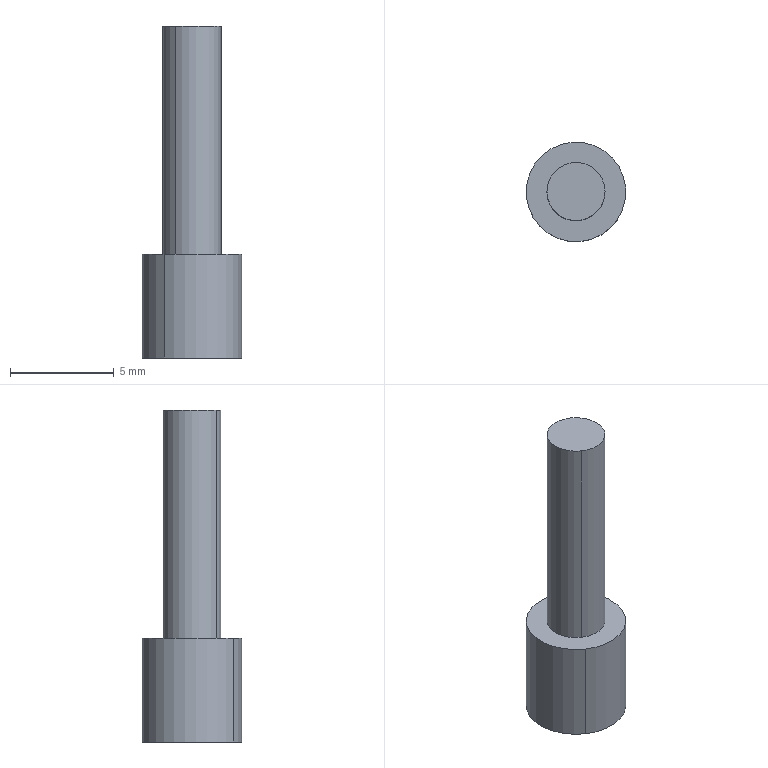Component | SolidWorks | F-YBXFJFA-RB0806-1_F-YBXFJFA-RB0806_Rb-Rod-1 | 1 solid | 7 faces | box 4.8 x 4.8 x 16 mm | volume 158 mm3 | cylinder 4 | plane 3 | commonest cylinder face diameters 4.8 x2 2.8 x2
build123d program:
from build123d import *

# Parameters (mm, degrees)
SKETCH1_R           = 1.4
BASE_EXTRUDE_DEPTH  = 11
SKETCH2_R           = 2.4
BOSS_EXTRUDE1_DEPTH = 5


with BuildPart() as part:
    # Sketch1 → Base-Extrude (new body)
    with BuildSketch(Plane.XY):
        Circle(SKETCH1_R)
    extrude(amount=BASE_EXTRUDE_DEPTH)

    # Sketch2 → Boss-Extrude1 (add)
    with BuildSketch(Plane(origin=(0, 0, 0), x_dir=(-1, 0, 0), z_dir=(0, 0, -1))):
        Circle(SKETCH2_R)
    extrude(amount=BOSS_EXTRUDE1_DEPTH)


solid = part.part

# Placed as in the assembly
solid = solid.moved(Location((272.305, 309.175, 63.479), (0, 0, 0)))
STEP:
#1=CARTESIAN_POINT('',(10.668,12.094,2.302));
#2=VERTEX_POINT('',#1);
#3=CARTESIAN_POINT('',(10.774,12.25,2.302));
#4=VERTEX_POINT('',#3);
#5=CARTESIAN_POINT('',(10.721,12.172,2.302));
#6=DIRECTION('',(0.,0.,-1.));
#7=DIRECTION('',(-0.5614,-0.8276,0.));
#8=AXIS2_PLACEMENT_3D('',#5,#6,#7);
#9=CIRCLE('',#8,0.09449);
#10=EDGE_CURVE('',#2,#4,#9,.T.);
#11=ORIENTED_EDGE('',*,*,#10,.F.);
#12=CARTESIAN_POINT('',(10.668,12.094,2.499));
#13=VERTEX_POINT('',#12);
#14=CARTESIAN_POINT('',(10.668,12.094,2.302));
#15=DIRECTION('',(0.,0.,1.));
#16=VECTOR('',#15,39.37);
#17=LINE('',#14,#16);
#18=EDGE_CURVE('',#2,#13,#17,.T.);
#19=ORIENTED_EDGE('',*,*,#18,.T.);
#20=CARTESIAN_POINT('',(10.774,12.25,2.499));
#21=VERTEX_POINT('',#20);
#22=CARTESIAN_POINT('',(10.721,12.172,2.499));
#23=DIRECTION('',(0.,0.,-1.));
#24=DIRECTION('',(-0.5614,-0.8276,0.));
#25=AXIS2_PLACEMENT_3D('',#22,#23,#24);
#26=CIRCLE('',#25,0.09449);
#27=EDGE_CURVE('',#13,#21,#26,.T.);
#28=ORIENTED_EDGE('',*,*,#27,.T.);
#29=CARTESIAN_POINT('',(10.774,12.25,2.302));
#30=DIRECTION('',(0.,0.,1.));
#31=VECTOR('',#30,39.37);
#32=LINE('',#29,#31);
#33=EDGE_CURVE('',#4,#21,#32,.T.);
#34=ORIENTED_EDGE('',*,*,#33,.F.);
#35=EDGE_LOOP('',(#11,#19,#28,#34));
#36=FACE_OUTER_BOUND('',#35,.T.);
#37=CARTESIAN_POINT('',(10.721,12.172,2.302));
#38=DIRECTION('',(0.,0.,1.));
#39=DIRECTION('',(0.5614,0.8276,0.));
#40=AXIS2_PLACEMENT_3D('',#37,#38,#39);
#41=CYLINDRICAL_SURFACE('',#40,0.09449);
#42=ADVANCED_FACE('',(#36),#41,.T.);
#43=CARTESIAN_POINT('',(10.752,12.218,2.932));
#44=VERTEX_POINT('',#43);
#45=CARTESIAN_POINT('',(10.69,12.127,2.932));
#46=VERTEX_POINT('',#45);
#47=CARTESIAN_POINT('',(10.721,12.172,2.932));
#48=DIRECTION('',(0.,0.,1.));
#49=DIRECTION('',(0.5614,0.8276,0.));
#50=AXIS2_PLACEMENT_3D('',#47,#48,#49);
#51=CIRCLE('',#50,0.05512);
#52=EDGE_CURVE('',#44,#46,#51,.T.);
#53=ORIENTED_EDGE('',*,*,#52,.F.);
#54=CARTESIAN_POINT('',(10.752,12.218,2.499));
#55=VERTEX_POINT('',#54);
#56=CARTESIAN_POINT('',(10.752,12.218,2.932));
#57=DIRECTION('',(0.,0.,-1.));
#58=VECTOR('',#57,39.37);
#59=LINE('',#56,#58);
#60=EDGE_CURVE('',#44,#55,#59,.T.);
#61=ORIENTED_EDGE('',*,*,#60,.T.);
#62=CARTESIAN_POINT('',(10.69,12.127,2.499));
#63=VERTEX_POINT('',#62);
#64=CARTESIAN_POINT('',(10.721,12.172,2.499));
#65=DIRECTION('',(0.,0.,-1.));
#66=DIRECTION('',(-0.5614,-0.8276,0.));
#67=AXIS2_PLACEMENT_3D('',#64,#65,#66);
#68=CIRCLE('',#67,0.05512);
#69=EDGE_CURVE('',#63,#55,#68,.T.);
#70=ORIENTED_EDGE('',*,*,#69,.F.);
#71=CARTESIAN_POINT('',(10.69,12.127,2.932));
#72=DIRECTION('',(0.,0.,-1.));
#73=VECTOR('',#72,39.37);
#74=LINE('',#71,#73);
#75=EDGE_CURVE('',#46,#63,#74,.T.);
#76=ORIENTED_EDGE('',*,*,#75,.F.);
#77=EDGE_LOOP('',(#53,#61,#70,#76));
#78=FACE_OUTER_BOUND('',#77,.T.);
#79=CARTESIAN_POINT('',(10.721,12.172,2.932));
#80=DIRECTION('',(0.,0.,-1.));
#81=DIRECTION('',(-0.5614,-0.8276,0.));
#82=AXIS2_PLACEMENT_3D('',#79,#80,#81);
#83=CYLINDRICAL_SURFACE('',#82,0.05512);
#84=ADVANCED_FACE('',(#78),#83,.T.);
#85=ORIENTED_EDGE('',*,*,#60,.F.);
#86=CARTESIAN_POINT('',(10.721,12.172,2.932));
#87=DIRECTION('',(0.,0.,1.));
#88=DIRECTION('',(0.5614,0.8276,0.));
#89=AXIS2_PLACEMENT_3D('',#86,#87,#88);
#90=CIRCLE('',#89,0.05512);
#91=EDGE_CURVE('',#46,#44,#90,.T.);
#92=ORIENTED_EDGE('',*,*,#91,.F.);
#93=ORIENTED_EDGE('',*,*,#75,.T.);
#94=CARTESIAN_POINT('',(10.721,12.172,2.499));
#95=DIRECTION('',(0.,0.,-1.));
#96=DIRECTION('',(-0.5614,-0.8276,0.));
#97=AXIS2_PLACEMENT_3D('',#94,#95,#96);
#98=CIRCLE('',#97,0.05512);
#99=EDGE_CURVE('',#55,#63,#98,.T.);
#100=ORIENTED_EDGE('',*,*,#99,.F.);
#101=EDGE_LOOP('',(#85,#92,#93,#100));
#102=FACE_OUTER_BOUND('',#101,.T.);
#103=CARTESIAN_POINT('',(10.721,12.172,2.932));
#104=DIRECTION('',(0.,0.,-1.));
#105=DIRECTION('',(-0.5614,-0.8276,0.));
#106=AXIS2_PLACEMENT_3D('',#103,#104,#105);
#107=CYLINDRICAL_SURFACE('',#106,0.05512);
#108=ADVANCED_FACE('',(#102),#107,.T.);
#109=ORIENTED_EDGE('',*,*,#91,.T.);
#110=ORIENTED_EDGE('',*,*,#52,.T.);
#111=EDGE_LOOP('',(#109,#110));
#112=FACE_OUTER_BOUND('',#111,.T.);
#113=CARTESIAN_POINT('',(10.721,12.172,2.932));
#114=DIRECTION('',(0.,0.,1.));
#115=DIRECTION('',(0.5614,0.8276,0.));
#116=AXIS2_PLACEMENT_3D('',#113,#114,#115);
#117=PLANE('',#116);
#118=ADVANCED_FACE('',(#112),#117,.T.);
#119=CARTESIAN_POINT('',(10.721,12.172,2.499));
#120=DIRECTION('',(0.,0.,-1.));
#121=DIRECTION('',(-0.5614,-0.8276,0.));
#122=AXIS2_PLACEMENT_3D('',#119,#120,#121);
#123=CIRCLE('',#122,0.09449);
#124=EDGE_CURVE('',#21,#13,#123,.T.);
#125=ORIENTED_EDGE('',*,*,#124,.F.);
#126=ORIENTED_EDGE('',*,*,#27,.F.);
#127=EDGE_LOOP('',(#125,#126));
#128=FACE_OUTER_BOUND('',#127,.T.);
#129=ORIENTED_EDGE('',*,*,#69,.T.);
#130=ORIENTED_EDGE('',*,*,#99,.T.);
#131=EDGE_LOOP('',(#129,#130));
#132=FACE_BOUND('',#131,.T.);
#133=CARTESIAN_POINT('',(10.721,12.172,2.499));
#134=DIRECTION('',(0.,0.,-1.));
#135=DIRECTION('',(-0.5614,-0.8276,0.));
#136=AXIS2_PLACEMENT_3D('',#133,#134,#135);
#137=PLANE('',#136);
#138=ADVANCED_FACE('',(#128,#132),#137,.F.);
#139=ORIENTED_EDGE('',*,*,#18,.F.);
#140=CARTESIAN_POINT('',(10.721,12.172,2.302));
#141=DIRECTION('',(0.,0.,-1.));
#142=DIRECTION('',(-0.5614,-0.8276,0.));
#143=AXIS2_PLACEMENT_3D('',#140,#141,#142);
#144=CIRCLE('',#143,0.09449);
#145=EDGE_CURVE('',#4,#2,#144,.T.);
#146=ORIENTED_EDGE('',*,*,#145,.F.);
#147=ORIENTED_EDGE('',*,*,#33,.T.);
#148=ORIENTED_EDGE('',*,*,#124,.T.);
#149=EDGE_LOOP('',(#139,#146,#147,#148));
#150=FACE_OUTER_BOUND('',#149,.T.);
#151=CARTESIAN_POINT('',(10.721,12.172,2.302));
#152=DIRECTION('',(0.,0.,1.));
#153=DIRECTION('',(0.5614,0.8276,0.));
#154=AXIS2_PLACEMENT_3D('',#151,#152,#153);
#155=CYLINDRICAL_SURFACE('',#154,0.09449);
#156=ADVANCED_FACE('',(#150),#155,.T.);
#157=ORIENTED_EDGE('',*,*,#145,.T.);
#158=ORIENTED_EDGE('',*,*,#10,.T.);
#159=EDGE_LOOP('',(#157,#158));
#160=FACE_OUTER_BOUND('',#159,.T.);
#161=CARTESIAN_POINT('',(10.721,12.172,2.302));
#162=DIRECTION('',(0.,0.,-1.));
#163=DIRECTION('',(-0.5614,-0.8276,0.));
#164=AXIS2_PLACEMENT_3D('',#161,#162,#163);
#165=PLANE('',#164);
#166=ADVANCED_FACE('',(#160),#165,.T.);
#167=CLOSED_SHELL('',(#42,#84,#108,#118,#138,#156,#166));
#168=MANIFOLD_SOLID_BREP('',#167);
#169=CARTESIAN_POINT('',(0.,0.,0.));
#170=DIRECTION('',(0.,0.,1.));
#171=DIRECTION('',(1.,0.,0.));
#172=AXIS2_PLACEMENT_3D('',#169,#170,#171);
#173=(LENGTH_UNIT()NAMED_UNIT(*)SI_UNIT($,.METRE.));
#174=LENGTH_MEASURE_WITH_UNIT(LENGTH_MEASURE(0.0254),#173);
#175=DIMENSIONAL_EXPONENTS(1.,0.,0.,0.,0.,0.,0.);
#176=(CONVERSION_BASED_UNIT('',#174)LENGTH_UNIT()NAMED_UNIT(#175));
#177=UNCERTAINTY_MEASURE_WITH_UNIT(LENGTH_MEASURE(0.00001),#176,'','');
#178=(NAMED_UNIT(*)PLANE_ANGLE_UNIT()SI_UNIT($,.RADIAN.));
#179=(NAMED_UNIT(*)SI_UNIT($,.STERADIAN.)SOLID_ANGLE_UNIT());
#180=(GEOMETRIC_REPRESENTATION_CONTEXT(3)GLOBAL_UNCERTAINTY_ASSIGNED_CONTEXT((#177))GLOBAL_UNIT_ASSIGNED_CONTEXT((#176,#178,#179))REPRESENTATION_CONTEXT('',''));
#181=ADVANCED_BREP_SHAPE_REPRESENTATION('',(#168,#172),#180);
#182=COLOUR_RGB('',0.7922,0.8196,0.9333);
#183=FILL_AREA_STYLE_COLOUR('',#182);
#184=FILL_AREA_STYLE('',(#183));
#185=SURFACE_STYLE_FILL_AREA(#184);
#186=SURFACE_SIDE_STYLE('',(#185));
#187=SURFACE_STYLE_USAGE(.BOTH.,#186);
#188=PRESENTATION_STYLE_ASSIGNMENT((#187));
#189=STYLED_ITEM('',(#188),#168);
#190=PRESENTATION_LAYER_ASSIGNMENT('','',(#189));
#191=(LENGTH_UNIT()NAMED_UNIT(*)SI_UNIT($,.METRE.));
#192=LENGTH_MEASURE_WITH_UNIT(LENGTH_MEASURE(0.0254),#191);
#193=DIMENSIONAL_EXPONENTS(1.,0.,0.,0.,0.,0.,0.);
#194=(CONVERSION_BASED_UNIT('',#192)LENGTH_UNIT()NAMED_UNIT(#193));
#195=UNCERTAINTY_MEASURE_WITH_UNIT(LENGTH_MEASURE(0.00001),#194,'','');
#196=(NAMED_UNIT(*)PLANE_ANGLE_UNIT()SI_UNIT($,.RADIAN.));
#197=(NAMED_UNIT(*)SI_UNIT($,.STERADIAN.)SOLID_ANGLE_UNIT());
#198=(GEOMETRIC_REPRESENTATION_CONTEXT(3)GLOBAL_UNCERTAINTY_ASSIGNED_CONTEXT((#195))GLOBAL_UNIT_ASSIGNED_CONTEXT((#194,#196,#197))REPRESENTATION_CONTEXT('',''));
#199=MECHANICAL_DESIGN_GEOMETRIC_PRESENTATION_REPRESENTATION('',(#189),#198);